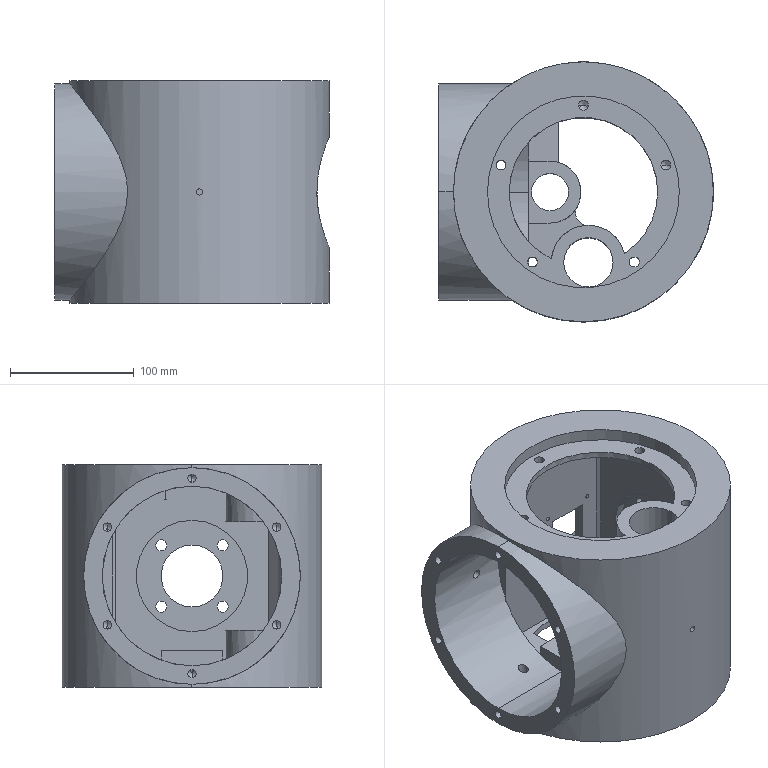Component | SolidWorks | 7-1 | 1 solid | 182 faces | volume 2588729 mm3 | cylinder 107 | plane 46 | cone 29 | commonest cylinder face diameters 8 x20 6.8 x14 3.3 x8 9 x8 14 x8 120 x5 10.2 x4 90 x4